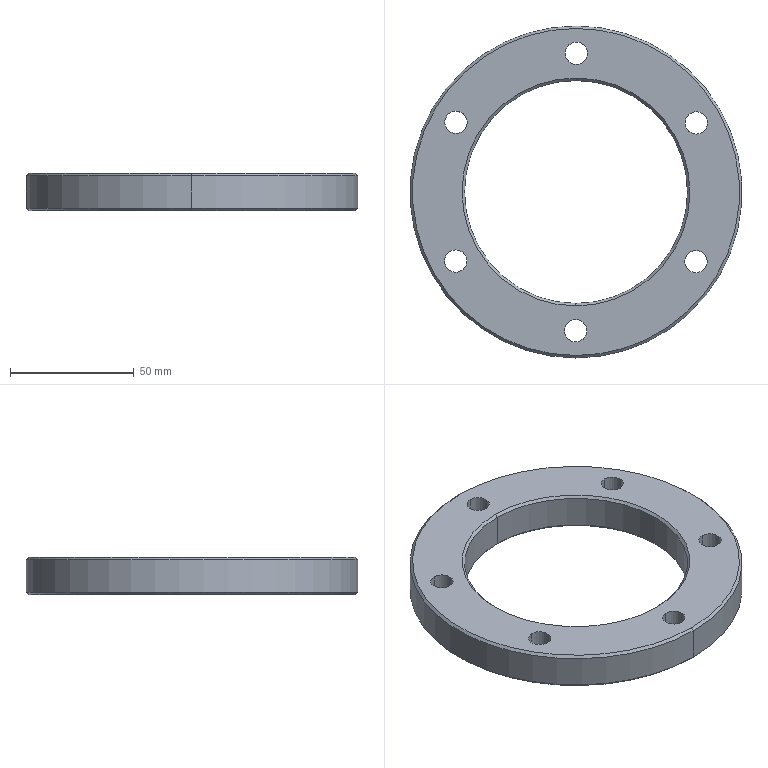Component | SolidWorks | ZN-A-027-1 | 1 solid | 44 faces | volume 103848 mm3 | cylinder 28 | cone 8 | plane 8 | commonest cylinder face diameters 15 x12 9 x12 90 x2 134 x2